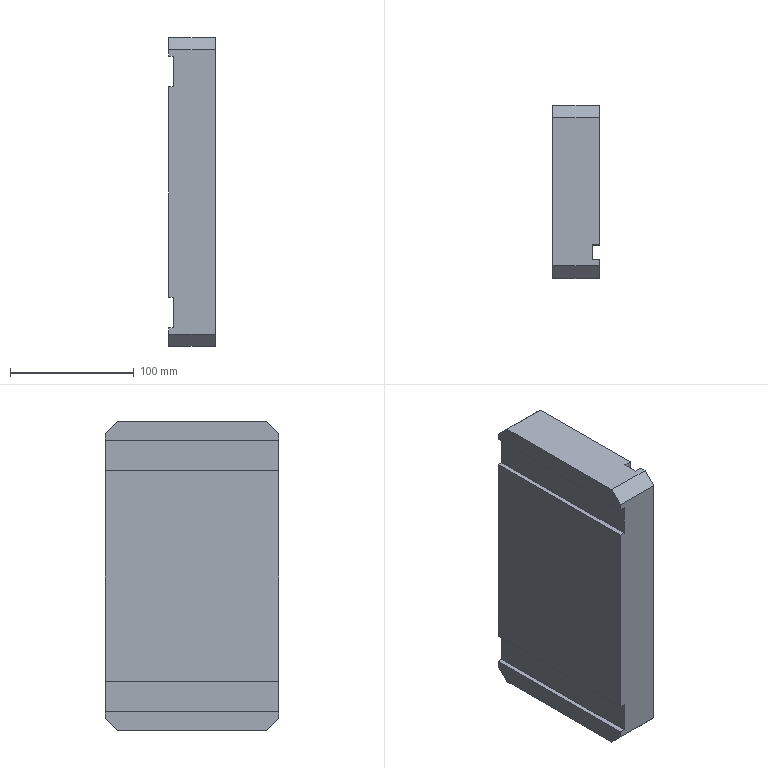Component | SolidWorks | 100-05-1 | 1 solid | 62 faces | box 38 x 140 x 250 mm | volume 1269662 mm3 | plane 22 | cylinder 20 | cone 20 | commonest cylinder face diameters 6.8 x16 2.5 x4 | material 45
build123d program:
from build123d import *

# Parameters (mm, degrees)
SKETCH1_W             = 140
SKETCH1_H             = 250
BOSS_EXTRUDE1_DEPTH   = 19
CHAMFER1_SIZE         = 10
SKETCH2_W             = 12
SKETCH2_H             = 250
CUT_EXTRUDE1_DEPTH    = 6
M8_TAPPED_HOLE1_D     = 6.8
M8_TAPPED_HOLE1_DEPTH = 23.75
M8_TAPPED_HOLE1_TIP   = 2.043
SKETCH5_W             = 140
SKETCH5_H             = 25
CUT_EXTRUDE2_DEPTH    = 4
M3_TAPPED_HOLE1_D     = 2.5
M3_TAPPED_HOLE1_DEPTH = 7.5
M3_TAPPED_HOLE1_TIP   = 0.7511


with BuildPart() as part:
    # Sketch1 → Boss-Extrude1 (new, symmetric)
    with BuildSketch(Plane(origin=(0, 0, 0), x_dir=(1, 0, 0), z_dir=(0, 1, 0))):
        Rectangle(SKETCH1_W, SKETCH1_H)
    extrude(amount=BOSS_EXTRUDE1_DEPTH, both=True)

    # Chamfer1
    chamfer1_edges = [part.edges().sort_by_distance(p)[0] for p in [
        (-70, 0, -125),
        (70, 0, -125),
        (70, 0, 125),
        (-70, 0, 125),
    ]]
    chamfer(chamfer1_edges, length=CHAMFER1_SIZE)

    # Sketch2 → Cut-Extrude1 (cut)
    with BuildSketch(Plane(origin=(0, 19, 0), x_dir=(1, 0, 0), z_dir=(0, 1, 0))):
        with Locations((-49, 0)):
            Rectangle(SKETCH2_W, SKETCH2_H)
    extrude(amount=-CUT_EXTRUDE1_DEPTH, mode=Mode.SUBTRACT)

    # M8 Tapped Hole1
    with Locations(Plane(origin=(0, 19, 0), x_dir=(1, 0, 0), z_dir=(0, 1, 0))):
        with Locations((31, 58), (31, -58), (-49, -58), (-49, 58), (-2, 110), (-30, 110), (-2, -110), (-30, -110)):
            Hole(M8_TAPPED_HOLE1_D / 2, depth=M8_TAPPED_HOLE1_DEPTH)
            with Locations((0, 0, -(M8_TAPPED_HOLE1_DEPTH + M8_TAPPED_HOLE1_TIP / 2))):  # 118° drill point
                Cone(0, M8_TAPPED_HOLE1_D / 2, M8_TAPPED_HOLE1_TIP, mode=Mode.SUBTRACT)

    # Sketch5 → Cut-Extrude2 (cut)
    with BuildSketch(Plane.XZ.offset(19)):
        with Locations((0, -97.5)):
            Rectangle(SKETCH5_W, SKETCH5_H)
    cut_extrude2 = extrude(amount=-CUT_EXTRUDE2_DEPTH, mode=Mode.SUBTRACT)

    # Mirror1: Cut-Extrude2 across plane
    add(cut_extrude2.mirror(Plane.XY), mode=Mode.SUBTRACT)

    # M3 Tapped Hole1
    with Locations(Plane.XY.offset(125)):
        with Locations((-50, 9), (-18, 9)):
            Hole(M3_TAPPED_HOLE1_D / 2, depth=M3_TAPPED_HOLE1_DEPTH)
            with Locations((0, 0, -(M3_TAPPED_HOLE1_DEPTH + M3_TAPPED_HOLE1_TIP / 2))):  # 118° drill point
                Cone(0, M3_TAPPED_HOLE1_D / 2, M3_TAPPED_HOLE1_TIP, mode=Mode.SUBTRACT)


solid = part.part

# Placed as in the assembly
solid = solid.moved(Location((160, 801, 0), (180, 0, -90)))